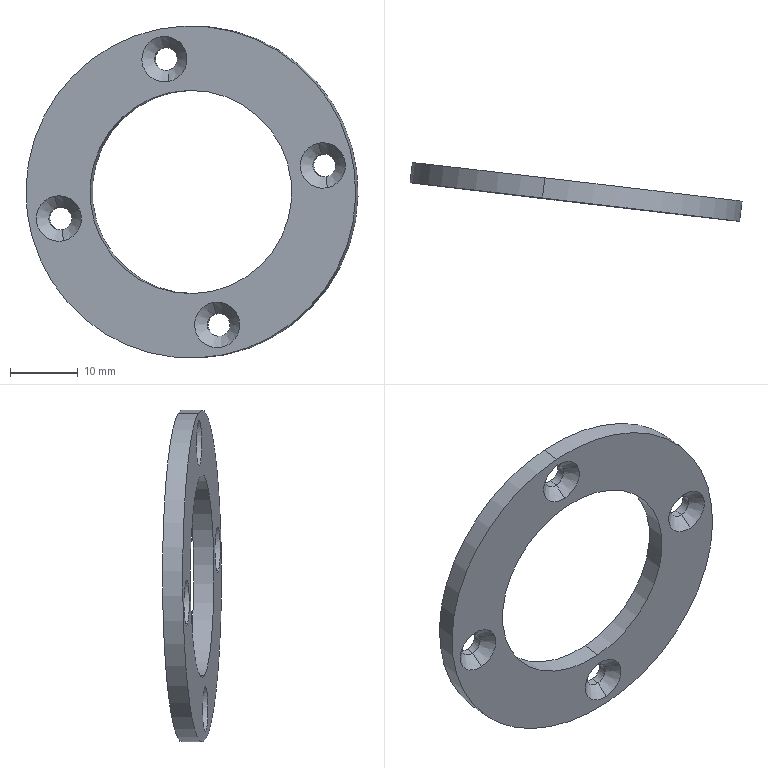Component | SolidWorks | 8TC-A17001-91-00UpperAndLowerPressAssembly-1_8TC-A17001-91-03Gland-1 | 1 solid | 22 faces | box 49.02 x 8.7 x 49 mm | volume 3350 mm3 | cylinder 12 | cone 8 | plane 2 | commonest cylinder face diameters 3.4 x8 30 x2 49 x2 | material A3
STEP:
#1=COLOUR_RGB('',0.7922,0.8196,0.9333);
#2=FILL_AREA_STYLE_COLOUR('',#1);
#3=FILL_AREA_STYLE('',(#2));
#4=SURFACE_STYLE_FILL_AREA(#3);
#5=SURFACE_SIDE_STYLE('',(#4));
#6=SURFACE_STYLE_USAGE(.BOTH.,#5);
#7=PRESENTATION_STYLE_ASSIGNMENT((#6));
#8=CARTESIAN_POINT('',(0.1834,-3.281,-2.754));
#9=VERTEX_POINT('',#8);
#10=CARTESIAN_POINT('',(0.2095,-3.284,-2.885));
#11=VERTEX_POINT('',#10);
#12=CARTESIAN_POINT('',(0.1964,-3.282,-2.819));
#13=DIRECTION('',(-0.1167,-0.9932,0.));
#14=DIRECTION('',(0.1946,-0.02286,-0.9806));
#15=AXIS2_PLACEMENT_3D('',#12,#13,#14);
#16=CIRCLE('',#15,0.06693);
#17=EDGE_CURVE('',#9,#11,#16,.T.);
#18=ORIENTED_EDGE('',*,*,#17,.F.);
#19=CARTESIAN_POINT('',(0.1631,-3.344,-2.69));
#20=VERTEX_POINT('',#19);
#21=CARTESIAN_POINT('',(0.1631,-3.344,-2.69));
#22=DIRECTION('',(-0.2201,-0.6861,0.6934));
#23=VECTOR('',#22,39.37);
#24=LINE('',#21,#23);
#25=EDGE_CURVE('',#9,#20,#24,.T.);
#26=ORIENTED_EDGE('',*,*,#25,.T.);
#27=CARTESIAN_POINT('',(0.2145,-3.35,-2.949));
#28=VERTEX_POINT('',#27);
#29=CARTESIAN_POINT('',(0.1888,-3.347,-2.819));
#30=DIRECTION('',(-0.1167,-0.9932,0.));
#31=DIRECTION('',(0.1946,-0.02286,-0.9806));
#32=AXIS2_PLACEMENT_3D('',#29,#30,#31);
#33=CIRCLE('',#32,0.1323);
#34=EDGE_CURVE('',#20,#28,#33,.T.);
#35=ORIENTED_EDGE('',*,*,#34,.T.);
#36=CARTESIAN_POINT('',(0.2145,-3.35,-2.949));
#37=DIRECTION('',(0.05511,-0.7184,-0.6934));
#38=VECTOR('',#37,39.37);
#39=LINE('',#36,#38);
#40=EDGE_CURVE('',#11,#28,#39,.T.);
#41=ORIENTED_EDGE('',*,*,#40,.F.);
#42=EDGE_LOOP('',(#18,#26,#35,#41));
#43=FACE_OUTER_BOUND('',#42,.T.);
#44=CARTESIAN_POINT('',(0.1888,-3.347,-2.819));
#45=DIRECTION('',(-0.1167,-0.9932,0.));
#46=DIRECTION('',(0.1946,-0.02286,-0.9806));
#47=AXIS2_PLACEMENT_3D('',#44,#45,#46);
#48=CONICAL_SURFACE('',#47,0.1323,0.7854);
#49=ADVANCED_FACE('',(#43),#48,.F.);
#50=CARTESIAN_POINT('',(0.1896,-3.228,-2.754));
#51=VERTEX_POINT('',#50);
#52=CARTESIAN_POINT('',(0.2156,-3.232,-2.885));
#53=VERTEX_POINT('',#52);
#54=CARTESIAN_POINT('',(0.2026,-3.23,-2.819));
#55=DIRECTION('',(-0.1167,-0.9932,0.));
#56=DIRECTION('',(0.1946,-0.02286,-0.9806));
#57=AXIS2_PLACEMENT_3D('',#54,#55,#56);
#58=CIRCLE('',#57,0.06693);
#59=EDGE_CURVE('',#51,#53,#58,.T.);
#60=ORIENTED_EDGE('',*,*,#59,.F.);
#61=CARTESIAN_POINT('',(0.1758,-3.346,-2.754));
#62=DIRECTION('',(-0.1167,-0.9932,0.));
#63=VECTOR('',#62,39.37);
#64=LINE('',#61,#63);
#65=EDGE_CURVE('',#51,#9,#64,.T.);
#66=ORIENTED_EDGE('',*,*,#65,.T.);
#67=ORIENTED_EDGE('',*,*,#17,.T.);
#68=CARTESIAN_POINT('',(0.2018,-3.349,-2.885));
#69=DIRECTION('',(-0.1167,-0.9932,0.));
#70=VECTOR('',#69,39.37);
#71=LINE('',#68,#70);
#72=EDGE_CURVE('',#53,#11,#71,.T.);
#73=ORIENTED_EDGE('',*,*,#72,.F.);
#74=EDGE_LOOP('',(#60,#66,#67,#73));
#75=FACE_OUTER_BOUND('',#74,.T.);
#76=CARTESIAN_POINT('',(0.1888,-3.347,-2.819));
#77=DIRECTION('',(-0.1167,-0.9932,0.));
#78=DIRECTION('',(0.1946,-0.02286,-0.9806));
#79=AXIS2_PLACEMENT_3D('',#76,#77,#78);
#80=CYLINDRICAL_SURFACE('',#79,0.06693);
#81=ADVANCED_FACE('',(#75),#80,.F.);
#82=CARTESIAN_POINT('',(0.797,-3.353,-1.827));
#83=VERTEX_POINT('',#82);
#84=CARTESIAN_POINT('',(0.8231,-3.356,-1.959));
#85=VERTEX_POINT('',#84);
#86=CARTESIAN_POINT('',(0.8101,-3.355,-1.893));
#87=DIRECTION('',(-0.1167,-0.9932,0.));
#88=DIRECTION('',(0.1946,-0.02286,-0.9806));
#89=AXIS2_PLACEMENT_3D('',#86,#87,#88);
#90=CIRCLE('',#89,0.06693);
#91=EDGE_CURVE('',#83,#85,#90,.T.);
#92=ORIENTED_EDGE('',*,*,#91,.F.);
#93=CARTESIAN_POINT('',(0.7767,-3.416,-1.763));
#94=VERTEX_POINT('',#93);
#95=CARTESIAN_POINT('',(0.7767,-3.416,-1.763));
#96=DIRECTION('',(-0.2201,-0.6861,0.6934));
#97=VECTOR('',#96,39.37);
#98=LINE('',#95,#97);
#99=EDGE_CURVE('',#83,#94,#98,.T.);
#100=ORIENTED_EDGE('',*,*,#99,.T.);
#101=CARTESIAN_POINT('',(0.8282,-3.422,-2.023));
#102=VERTEX_POINT('',#101);
#103=CARTESIAN_POINT('',(0.8024,-3.419,-1.893));
#104=DIRECTION('',(-0.1167,-0.9932,0.));
#105=DIRECTION('',(0.1946,-0.02286,-0.9806));
#106=AXIS2_PLACEMENT_3D('',#103,#104,#105);
#107=CIRCLE('',#106,0.1323);
#108=EDGE_CURVE('',#94,#102,#107,.T.);
#109=ORIENTED_EDGE('',*,*,#108,.T.);
#110=CARTESIAN_POINT('',(0.8282,-3.422,-2.023));
#111=DIRECTION('',(0.05511,-0.7184,-0.6934));
#112=VECTOR('',#111,39.37);
#113=LINE('',#110,#112);
#114=EDGE_CURVE('',#85,#102,#113,.T.);
#115=ORIENTED_EDGE('',*,*,#114,.F.);
#116=EDGE_LOOP('',(#92,#100,#109,#115));
#117=FACE_OUTER_BOUND('',#116,.T.);
#118=CARTESIAN_POINT('',(0.8024,-3.419,-1.893));
#119=DIRECTION('',(-0.1167,-0.9932,0.));
#120=DIRECTION('',(0.1946,-0.02286,-0.9806));
#121=AXIS2_PLACEMENT_3D('',#118,#119,#120);
#122=CONICAL_SURFACE('',#121,0.1323,0.7854);
#123=ADVANCED_FACE('',(#117),#122,.F.);
#124=CARTESIAN_POINT('',(0.8032,-3.301,-1.827));
#125=VERTEX_POINT('',#124);
#126=CARTESIAN_POINT('',(0.8292,-3.304,-1.959));
#127=VERTEX_POINT('',#126);
#128=CARTESIAN_POINT('',(0.8162,-3.302,-1.893));
#129=DIRECTION('',(-0.1167,-0.9932,0.));
#130=DIRECTION('',(0.1946,-0.02286,-0.9806));
#131=AXIS2_PLACEMENT_3D('',#128,#129,#130);
#132=CIRCLE('',#131,0.06693);
#133=EDGE_CURVE('',#125,#127,#132,.T.);
#134=ORIENTED_EDGE('',*,*,#133,.F.);
#135=CARTESIAN_POINT('',(0.7894,-3.418,-1.827));
#136=DIRECTION('',(-0.1167,-0.9932,0.));
#137=VECTOR('',#136,39.37);
#138=LINE('',#135,#137);
#139=EDGE_CURVE('',#125,#83,#138,.T.);
#140=ORIENTED_EDGE('',*,*,#139,.T.);
#141=ORIENTED_EDGE('',*,*,#91,.T.);
#142=CARTESIAN_POINT('',(0.8155,-3.421,-1.959));
#143=DIRECTION('',(-0.1167,-0.9932,0.));
#144=VECTOR('',#143,39.37);
#145=LINE('',#142,#144);
#146=EDGE_CURVE('',#127,#85,#145,.T.);
#147=ORIENTED_EDGE('',*,*,#146,.F.);
#148=EDGE_LOOP('',(#134,#140,#141,#147));
#149=FACE_OUTER_BOUND('',#148,.T.);
#150=CARTESIAN_POINT('',(0.8024,-3.419,-1.893));
#151=DIRECTION('',(-0.1167,-0.9932,0.));
#152=DIRECTION('',(0.1946,-0.02286,-0.9806));
#153=AXIS2_PLACEMENT_3D('',#150,#151,#152);
#154=CYLINDRICAL_SURFACE('',#153,0.06693);
#155=ADVANCED_FACE('',(#149),#154,.F.);
#156=CARTESIAN_POINT('',(-0.1231,-3.245,-1.209));
#157=VERTEX_POINT('',#156);
#158=CARTESIAN_POINT('',(-0.09702,-3.248,-1.341));
#159=VERTEX_POINT('',#158);
#160=CARTESIAN_POINT('',(-0.11,-3.246,-1.275));
#161=DIRECTION('',(-0.1167,-0.9932,0.));
#162=DIRECTION('',(0.1946,-0.02286,-0.9806));
#163=AXIS2_PLACEMENT_3D('',#160,#161,#162);
#164=CIRCLE('',#163,0.06693);
#165=EDGE_CURVE('',#157,#159,#164,.T.);
#166=ORIENTED_EDGE('',*,*,#165,.F.);
#167=CARTESIAN_POINT('',(-0.1434,-3.308,-1.145));
#168=VERTEX_POINT('',#167);
#169=CARTESIAN_POINT('',(-0.1434,-3.308,-1.145));
#170=DIRECTION('',(-0.2201,-0.6861,0.6934));
#171=VECTOR('',#170,39.37);
#172=LINE('',#169,#171);
#173=EDGE_CURVE('',#157,#168,#172,.T.);
#174=ORIENTED_EDGE('',*,*,#173,.T.);
#175=CARTESIAN_POINT('',(-0.09192,-3.314,-1.405));
#176=VERTEX_POINT('',#175);
#177=CARTESIAN_POINT('',(-0.1177,-3.311,-1.275));
#178=DIRECTION('',(-0.1167,-0.9932,0.));
#179=DIRECTION('',(0.1946,-0.02286,-0.9806));
#180=AXIS2_PLACEMENT_3D('',#177,#178,#179);
#181=CIRCLE('',#180,0.1323);
#182=EDGE_CURVE('',#168,#176,#181,.T.);
#183=ORIENTED_EDGE('',*,*,#182,.T.);
#184=CARTESIAN_POINT('',(-0.09192,-3.314,-1.405));
#185=DIRECTION('',(0.05511,-0.7184,-0.6934));
#186=VECTOR('',#185,39.37);
#187=LINE('',#184,#186);
#188=EDGE_CURVE('',#159,#176,#187,.T.);
#189=ORIENTED_EDGE('',*,*,#188,.F.);
#190=EDGE_LOOP('',(#166,#174,#183,#189));
#191=FACE_OUTER_BOUND('',#190,.T.);
#192=CARTESIAN_POINT('',(-0.1177,-3.311,-1.275));
#193=DIRECTION('',(-0.1167,-0.9932,0.));
#194=DIRECTION('',(0.1946,-0.02286,-0.9806));
#195=AXIS2_PLACEMENT_3D('',#192,#193,#194);
#196=CONICAL_SURFACE('',#195,0.1323,0.7854);
#197=ADVANCED_FACE('',(#191),#196,.F.);
#198=CARTESIAN_POINT('',(-0.1169,-3.192,-1.209));
#199=VERTEX_POINT('',#198);
#200=CARTESIAN_POINT('',(-0.09086,-3.196,-1.341));
#201=VERTEX_POINT('',#200);
#202=CARTESIAN_POINT('',(-0.1039,-3.194,-1.275));
#203=DIRECTION('',(-0.1167,-0.9932,0.));
#204=DIRECTION('',(0.1946,-0.02286,-0.9806));
#205=AXIS2_PLACEMENT_3D('',#202,#203,#204);
#206=CIRCLE('',#205,0.06693);
#207=EDGE_CURVE('',#199,#201,#206,.T.);
#208=ORIENTED_EDGE('',*,*,#207,.F.);
#209=CARTESIAN_POINT('',(-0.1307,-3.31,-1.209));
#210=DIRECTION('',(-0.1167,-0.9932,0.));
#211=VECTOR('',#210,39.37);
#212=LINE('',#209,#211);
#213=EDGE_CURVE('',#199,#157,#212,.T.);
#214=ORIENTED_EDGE('',*,*,#213,.T.);
#215=ORIENTED_EDGE('',*,*,#165,.T.);
#216=CARTESIAN_POINT('',(-0.1046,-3.313,-1.341));
#217=DIRECTION('',(-0.1167,-0.9932,0.));
#218=VECTOR('',#217,39.37);
#219=LINE('',#216,#218);
#220=EDGE_CURVE('',#201,#159,#219,.T.);
#221=ORIENTED_EDGE('',*,*,#220,.F.);
#222=EDGE_LOOP('',(#208,#214,#215,#221));
#223=FACE_OUTER_BOUND('',#222,.T.);
#224=CARTESIAN_POINT('',(-0.1177,-3.311,-1.275));
#225=DIRECTION('',(-0.1167,-0.9932,0.));
#226=DIRECTION('',(0.1946,-0.02286,-0.9806));
#227=AXIS2_PLACEMENT_3D('',#224,#225,#226);
#228=CYLINDRICAL_SURFACE('',#227,0.06693);
#229=ADVANCED_FACE('',(#223),#228,.F.);
#230=CARTESIAN_POINT('',(-0.7367,-3.173,-2.136));
#231=VERTEX_POINT('',#230);
#232=CARTESIAN_POINT('',(-0.7106,-3.176,-2.267));
#233=VERTEX_POINT('',#232);
#234=CARTESIAN_POINT('',(-0.7237,-3.174,-2.202));
#235=DIRECTION('',(-0.1167,-0.9932,0.));
#236=DIRECTION('',(0.1946,-0.02286,-0.9806));
#237=AXIS2_PLACEMENT_3D('',#234,#235,#236);
#238=CIRCLE('',#237,0.06693);
#239=EDGE_CURVE('',#231,#233,#238,.T.);
#240=ORIENTED_EDGE('',*,*,#239,.F.);
#241=CARTESIAN_POINT('',(-0.757,-3.236,-2.072));
#242=VERTEX_POINT('',#241);
#243=CARTESIAN_POINT('',(-0.757,-3.236,-2.072));
#244=DIRECTION('',(-0.2201,-0.6861,0.6934));
#245=VECTOR('',#244,39.37);
#246=LINE('',#243,#245);
#247=EDGE_CURVE('',#231,#242,#246,.T.);
#248=ORIENTED_EDGE('',*,*,#247,.T.);
#249=CARTESIAN_POINT('',(-0.7056,-3.242,-2.331));
#250=VERTEX_POINT('',#249);
#251=CARTESIAN_POINT('',(-0.7313,-3.239,-2.202));
#252=DIRECTION('',(-0.1167,-0.9932,0.));
#253=DIRECTION('',(0.1946,-0.02286,-0.9806));
#254=AXIS2_PLACEMENT_3D('',#251,#252,#253);
#255=CIRCLE('',#254,0.1323);
#256=EDGE_CURVE('',#242,#250,#255,.T.);
#257=ORIENTED_EDGE('',*,*,#256,.T.);
#258=CARTESIAN_POINT('',(-0.7056,-3.242,-2.331));
#259=DIRECTION('',(0.05511,-0.7184,-0.6934));
#260=VECTOR('',#259,39.37);
#261=LINE('',#258,#260);
#262=EDGE_CURVE('',#233,#250,#261,.T.);
#263=ORIENTED_EDGE('',*,*,#262,.F.);
#264=EDGE_LOOP('',(#240,#248,#257,#263));
#265=FACE_OUTER_BOUND('',#264,.T.);
#266=CARTESIAN_POINT('',(-0.7313,-3.239,-2.202));
#267=DIRECTION('',(-0.1167,-0.9932,0.));
#268=DIRECTION('',(0.1946,-0.02286,-0.9806));
#269=AXIS2_PLACEMENT_3D('',#266,#267,#268);
#270=CONICAL_SURFACE('',#269,0.1323,0.7854);
#271=ADVANCED_FACE('',(#265),#270,.F.);
#272=CARTESIAN_POINT('',(-0.7305,-3.12,-2.136));
#273=VERTEX_POINT('',#272);
#274=CARTESIAN_POINT('',(-0.7045,-3.123,-2.267));
#275=VERTEX_POINT('',#274);
#276=CARTESIAN_POINT('',(-0.7175,-3.122,-2.202));
#277=DIRECTION('',(-0.1167,-0.9932,0.));
#278=DIRECTION('',(0.1946,-0.02286,-0.9806));
#279=AXIS2_PLACEMENT_3D('',#276,#277,#278);
#280=CIRCLE('',#279,0.06693);
#281=EDGE_CURVE('',#273,#275,#280,.T.);
#282=ORIENTED_EDGE('',*,*,#281,.F.);
#283=CARTESIAN_POINT('',(-0.7443,-3.238,-2.136));
#284=DIRECTION('',(-0.1167,-0.9932,0.));
#285=VECTOR('',#284,39.37);
#286=LINE('',#283,#285);
#287=EDGE_CURVE('',#273,#231,#286,.T.);
#288=ORIENTED_EDGE('',*,*,#287,.T.);
#289=ORIENTED_EDGE('',*,*,#239,.T.);
#290=CARTESIAN_POINT('',(-0.7183,-3.241,-2.267));
#291=DIRECTION('',(-0.1167,-0.9932,0.));
#292=VECTOR('',#291,39.37);
#293=LINE('',#290,#292);
#294=EDGE_CURVE('',#275,#233,#293,.T.);
#295=ORIENTED_EDGE('',*,*,#294,.F.);
#296=EDGE_LOOP('',(#282,#288,#289,#295));
#297=FACE_OUTER_BOUND('',#296,.T.);
#298=CARTESIAN_POINT('',(-0.7313,-3.239,-2.202));
#299=DIRECTION('',(-0.1167,-0.9932,0.));
#300=DIRECTION('',(0.1946,-0.02286,-0.9806));
#301=AXIS2_PLACEMENT_3D('',#298,#299,#300);
#302=CYLINDRICAL_SURFACE('',#301,0.06693);
#303=ADVANCED_FACE('',(#297),#302,.F.);
#304=CARTESIAN_POINT('',(0.1643,-3.226,-2.626));
#305=VERTEX_POINT('',#304);
#306=CARTESIAN_POINT('',(-0.06558,-3.199,-1.468));
#307=VERTEX_POINT('',#306);
#308=CARTESIAN_POINT('',(0.04935,-3.212,-2.047));
#309=DIRECTION('',(0.1167,0.9932,-0.));
#310=DIRECTION('',(-0.1946,0.02286,0.9806));
#311=AXIS2_PLACEMENT_3D('',#308,#309,#310);
#312=CIRCLE('',#311,0.5906);
#313=EDGE_CURVE('',#305,#307,#312,.T.);
#314=ORIENTED_EDGE('',*,*,#313,.T.);
#315=CARTESIAN_POINT('',(-0.07936,-3.316,-1.468));
#316=VERTEX_POINT('',#315);
#317=CARTESIAN_POINT('',(-0.06558,-3.199,-1.468));
#318=DIRECTION('',(-0.1167,-0.9932,0.));
#319=VECTOR('',#318,39.37);
#320=LINE('',#317,#319);
#321=EDGE_CURVE('',#307,#316,#320,.T.);
#322=ORIENTED_EDGE('',*,*,#321,.T.);
#323=CARTESIAN_POINT('',(0.1505,-3.343,-2.626));
#324=VERTEX_POINT('',#323);
#325=CARTESIAN_POINT('',(0.03557,-3.329,-2.047));
#326=DIRECTION('',(0.1167,0.9932,-0.));
#327=DIRECTION('',(-0.1946,0.02286,0.9806));
#328=AXIS2_PLACEMENT_3D('',#325,#326,#327);
#329=CIRCLE('',#328,0.5906);
#330=EDGE_CURVE('',#324,#316,#329,.T.);
#331=ORIENTED_EDGE('',*,*,#330,.F.);
#332=CARTESIAN_POINT('',(0.1643,-3.226,-2.626));
#333=DIRECTION('',(-0.1167,-0.9932,0.));
#334=VECTOR('',#333,39.37);
#335=LINE('',#332,#334);
#336=EDGE_CURVE('',#305,#324,#335,.T.);
#337=ORIENTED_EDGE('',*,*,#336,.F.);
#338=EDGE_LOOP('',(#314,#322,#331,#337));
#339=FACE_OUTER_BOUND('',#338,.T.);
#340=CARTESIAN_POINT('',(0.04935,-3.212,-2.047));
#341=DIRECTION('',(-0.1167,-0.9932,0.));
#342=DIRECTION('',(0.1946,-0.02286,-0.9806));
#343=AXIS2_PLACEMENT_3D('',#340,#341,#342);
#344=CYLINDRICAL_SURFACE('',#343,0.5906);
#345=ADVANCED_FACE('',(#339),#344,.F.);
#346=CARTESIAN_POINT('',(-0.1384,-3.19,-1.101));
#347=VERTEX_POINT('',#346);
#348=CARTESIAN_POINT('',(0.2371,-3.234,-2.993));
#349=VERTEX_POINT('',#348);
#350=CARTESIAN_POINT('',(0.04935,-3.212,-2.047));
#351=DIRECTION('',(0.1167,0.9932,-0.));
#352=DIRECTION('',(-0.1946,0.02286,0.9806));
#353=AXIS2_PLACEMENT_3D('',#350,#351,#352);
#354=CIRCLE('',#353,0.9646);
#355=EDGE_CURVE('',#347,#349,#354,.T.);
#356=ORIENTED_EDGE('',*,*,#355,.F.);
#357=CARTESIAN_POINT('',(-0.1521,-3.307,-1.101));
#358=VERTEX_POINT('',#357);
#359=CARTESIAN_POINT('',(-0.1384,-3.19,-1.101));
#360=DIRECTION('',(-0.1167,-0.9932,0.));
#361=VECTOR('',#360,39.37);
#362=LINE('',#359,#361);
#363=EDGE_CURVE('',#347,#358,#362,.T.);
#364=ORIENTED_EDGE('',*,*,#363,.T.);
#365=CARTESIAN_POINT('',(0.2233,-3.351,-2.993));
#366=VERTEX_POINT('',#365);
#367=CARTESIAN_POINT('',(0.03557,-3.329,-2.047));
#368=DIRECTION('',(0.1167,0.9932,-0.));
#369=DIRECTION('',(-0.1946,0.02286,0.9806));
#370=AXIS2_PLACEMENT_3D('',#367,#368,#369);
#371=CIRCLE('',#370,0.9646);
#372=EDGE_CURVE('',#358,#366,#371,.T.);
#373=ORIENTED_EDGE('',*,*,#372,.T.);
#374=CARTESIAN_POINT('',(0.2371,-3.234,-2.993));
#375=DIRECTION('',(-0.1167,-0.9932,0.));
#376=VECTOR('',#375,39.37);
#377=LINE('',#374,#376);
#378=EDGE_CURVE('',#349,#366,#377,.T.);
#379=ORIENTED_EDGE('',*,*,#378,.F.);
#380=EDGE_LOOP('',(#356,#364,#373,#379));
#381=FACE_OUTER_BOUND('',#380,.T.);
#382=CARTESIAN_POINT('',(0.04935,-3.212,-2.047));
#383=DIRECTION('',(-0.1167,-0.9932,0.));
#384=DIRECTION('',(0.1946,-0.02286,-0.9806));
#385=AXIS2_PLACEMENT_3D('',#382,#383,#384);
#386=CYLINDRICAL_SURFACE('',#385,0.9646);
#387=ADVANCED_FACE('',(#381),#386,.T.);
#388=CARTESIAN_POINT('',(0.2026,-3.23,-2.819));
#389=DIRECTION('',(-0.1167,-0.9932,0.));
#390=DIRECTION('',(0.1946,-0.02286,-0.9806));
#391=AXIS2_PLACEMENT_3D('',#388,#389,#390);
#392=CIRCLE('',#391,0.06693);
#393=EDGE_CURVE('',#53,#51,#392,.T.);
#394=ORIENTED_EDGE('',*,*,#393,.T.);
#395=ORIENTED_EDGE('',*,*,#59,.T.);
#396=EDGE_LOOP('',(#394,#395));
#397=FACE_BOUND('',#396,.T.);
#398=CARTESIAN_POINT('',(0.8162,-3.302,-1.893));
#399=DIRECTION('',(-0.1167,-0.9932,0.));
#400=DIRECTION('',(0.1946,-0.02286,-0.9806));
#401=AXIS2_PLACEMENT_3D('',#398,#399,#400);
#402=CIRCLE('',#401,0.06693);
#403=EDGE_CURVE('',#127,#125,#402,.T.);
#404=ORIENTED_EDGE('',*,*,#403,.T.);
#405=ORIENTED_EDGE('',*,*,#133,.T.);
#406=EDGE_LOOP('',(#404,#405));
#407=FACE_BOUND('',#406,.T.);
#408=CARTESIAN_POINT('',(-0.1039,-3.194,-1.275));
#409=DIRECTION('',(-0.1167,-0.9932,0.));
#410=DIRECTION('',(0.1946,-0.02286,-0.9806));
#411=AXIS2_PLACEMENT_3D('',#408,#409,#410);
#412=CIRCLE('',#411,0.06693);
#413=EDGE_CURVE('',#201,#199,#412,.T.);
#414=ORIENTED_EDGE('',*,*,#413,.T.);
#415=ORIENTED_EDGE('',*,*,#207,.T.);
#416=EDGE_LOOP('',(#414,#415));
#417=FACE_BOUND('',#416,.T.);
#418=CARTESIAN_POINT('',(-0.7175,-3.122,-2.202));
#419=DIRECTION('',(-0.1167,-0.9932,0.));
#420=DIRECTION('',(0.1946,-0.02286,-0.9806));
#421=AXIS2_PLACEMENT_3D('',#418,#419,#420);
#422=CIRCLE('',#421,0.06693);
#423=EDGE_CURVE('',#275,#273,#422,.T.);
#424=ORIENTED_EDGE('',*,*,#423,.T.);
#425=ORIENTED_EDGE('',*,*,#281,.T.);
#426=EDGE_LOOP('',(#424,#425));
#427=FACE_BOUND('',#426,.T.);
#428=CARTESIAN_POINT('',(0.04935,-3.212,-2.047));
#429=DIRECTION('',(0.1167,0.9932,-0.));
#430=DIRECTION('',(-0.1946,0.02286,0.9806));
#431=AXIS2_PLACEMENT_3D('',#428,#429,#430);
#432=CIRCLE('',#431,0.9646);
#433=EDGE_CURVE('',#349,#347,#432,.T.);
#434=ORIENTED_EDGE('',*,*,#433,.T.);
#435=ORIENTED_EDGE('',*,*,#355,.T.);
#436=EDGE_LOOP('',(#434,#435));
#437=FACE_OUTER_BOUND('',#436,.T.);
#438=ORIENTED_EDGE('',*,*,#313,.F.);
#439=CARTESIAN_POINT('',(0.04935,-3.212,-2.047));
#440=DIRECTION('',(0.1167,0.9932,-0.));
#441=DIRECTION('',(-0.1946,0.02286,0.9806));
#442=AXIS2_PLACEMENT_3D('',#439,#440,#441);
#443=CIRCLE('',#442,0.5906);
#444=EDGE_CURVE('',#307,#305,#443,.T.);
#445=ORIENTED_EDGE('',*,*,#444,.F.);
#446=EDGE_LOOP('',(#438,#445));
#447=FACE_BOUND('',#446,.T.);
#448=CARTESIAN_POINT('',(0.04935,-3.212,-2.047));
#449=DIRECTION('',(0.1167,0.9932,-0.));
#450=DIRECTION('',(-0.1946,0.02286,0.9806));
#451=AXIS2_PLACEMENT_3D('',#448,#449,#450);
#452=PLANE('',#451);
#453=ADVANCED_FACE('',(#397,#407,#417,#427,#437,#447),#452,.T.);
#454=CARTESIAN_POINT('',(0.1888,-3.347,-2.819));
#455=DIRECTION('',(-0.1167,-0.9932,0.));
#456=DIRECTION('',(0.1946,-0.02286,-0.9806));
#457=AXIS2_PLACEMENT_3D('',#454,#455,#456);
#458=CIRCLE('',#457,0.1323);
#459=EDGE_CURVE('',#28,#20,#458,.T.);
#460=ORIENTED_EDGE('',*,*,#459,.F.);
#461=ORIENTED_EDGE('',*,*,#34,.F.);
#462=EDGE_LOOP('',(#460,#461));
#463=FACE_BOUND('',#462,.T.);
#464=CARTESIAN_POINT('',(0.8024,-3.419,-1.893));
#465=DIRECTION('',(-0.1167,-0.9932,0.));
#466=DIRECTION('',(0.1946,-0.02286,-0.9806));
#467=AXIS2_PLACEMENT_3D('',#464,#465,#466);
#468=CIRCLE('',#467,0.1323);
#469=EDGE_CURVE('',#102,#94,#468,.T.);
#470=ORIENTED_EDGE('',*,*,#469,.F.);
#471=ORIENTED_EDGE('',*,*,#108,.F.);
#472=EDGE_LOOP('',(#470,#471));
#473=FACE_BOUND('',#472,.T.);
#474=CARTESIAN_POINT('',(-0.1177,-3.311,-1.275));
#475=DIRECTION('',(-0.1167,-0.9932,0.));
#476=DIRECTION('',(0.1946,-0.02286,-0.9806));
#477=AXIS2_PLACEMENT_3D('',#474,#475,#476);
#478=CIRCLE('',#477,0.1323);
#479=EDGE_CURVE('',#176,#168,#478,.T.);
#480=ORIENTED_EDGE('',*,*,#479,.F.);
#481=ORIENTED_EDGE('',*,*,#182,.F.);
#482=EDGE_LOOP('',(#480,#481));
#483=FACE_BOUND('',#482,.T.);
#484=CARTESIAN_POINT('',(-0.7313,-3.239,-2.202));
#485=DIRECTION('',(-0.1167,-0.9932,0.));
#486=DIRECTION('',(0.1946,-0.02286,-0.9806));
#487=AXIS2_PLACEMENT_3D('',#484,#485,#486);
#488=CIRCLE('',#487,0.1323);
#489=EDGE_CURVE('',#250,#242,#488,.T.);
#490=ORIENTED_EDGE('',*,*,#489,.F.);
#491=ORIENTED_EDGE('',*,*,#256,.F.);
#492=EDGE_LOOP('',(#490,#491));
#493=FACE_BOUND('',#492,.T.);
#494=CARTESIAN_POINT('',(0.03557,-3.329,-2.047));
#495=DIRECTION('',(0.1167,0.9932,-0.));
#496=DIRECTION('',(-0.1946,0.02286,0.9806));
#497=AXIS2_PLACEMENT_3D('',#494,#495,#496);
#498=CIRCLE('',#497,0.9646);
#499=EDGE_CURVE('',#366,#358,#498,.T.);
#500=ORIENTED_EDGE('',*,*,#499,.F.);
#501=ORIENTED_EDGE('',*,*,#372,.F.);
#502=EDGE_LOOP('',(#500,#501));
#503=FACE_OUTER_BOUND('',#502,.T.);
#504=ORIENTED_EDGE('',*,*,#330,.T.);
#505=CARTESIAN_POINT('',(0.03557,-3.329,-2.047));
#506=DIRECTION('',(0.1167,0.9932,-0.));
#507=DIRECTION('',(-0.1946,0.02286,0.9806));
#508=AXIS2_PLACEMENT_3D('',#505,#506,#507);
#509=CIRCLE('',#508,0.5906);
#510=EDGE_CURVE('',#316,#324,#509,.T.);
#511=ORIENTED_EDGE('',*,*,#510,.T.);
#512=EDGE_LOOP('',(#504,#511));
#513=FACE_BOUND('',#512,.T.);
#514=CARTESIAN_POINT('',(0.03557,-3.329,-2.047));
#515=DIRECTION('',(0.1167,0.9932,-0.));
#516=DIRECTION('',(-0.1946,0.02286,0.9806));
#517=AXIS2_PLACEMENT_3D('',#514,#515,#516);
#518=PLANE('',#517);
#519=ADVANCED_FACE('',(#463,#473,#483,#493,#503,#513),#518,.F.);
#520=ORIENTED_EDGE('',*,*,#363,.F.);
#521=ORIENTED_EDGE('',*,*,#433,.F.);
#522=ORIENTED_EDGE('',*,*,#378,.T.);
#523=ORIENTED_EDGE('',*,*,#499,.T.);
#524=EDGE_LOOP('',(#520,#521,#522,#523));
#525=FACE_OUTER_BOUND('',#524,.T.);
#526=CARTESIAN_POINT('',(0.04935,-3.212,-2.047));
#527=DIRECTION('',(-0.1167,-0.9932,0.));
#528=DIRECTION('',(0.1946,-0.02286,-0.9806));
#529=AXIS2_PLACEMENT_3D('',#526,#527,#528);
#530=CYLINDRICAL_SURFACE('',#529,0.9646);
#531=ADVANCED_FACE('',(#525),#530,.T.);
#532=ORIENTED_EDGE('',*,*,#321,.F.);
#533=ORIENTED_EDGE('',*,*,#444,.T.);
#534=ORIENTED_EDGE('',*,*,#336,.T.);
#535=ORIENTED_EDGE('',*,*,#510,.F.);
#536=EDGE_LOOP('',(#532,#533,#534,#535));
#537=FACE_OUTER_BOUND('',#536,.T.);
#538=CARTESIAN_POINT('',(0.04935,-3.212,-2.047));
#539=DIRECTION('',(-0.1167,-0.9932,0.));
#540=DIRECTION('',(0.1946,-0.02286,-0.9806));
#541=AXIS2_PLACEMENT_3D('',#538,#539,#540);
#542=CYLINDRICAL_SURFACE('',#541,0.5906);
#543=ADVANCED_FACE('',(#537),#542,.F.);
#544=ORIENTED_EDGE('',*,*,#287,.F.);
#545=ORIENTED_EDGE('',*,*,#423,.F.);
#546=ORIENTED_EDGE('',*,*,#294,.T.);
#547=CARTESIAN_POINT('',(-0.7237,-3.174,-2.202));
#548=DIRECTION('',(-0.1167,-0.9932,0.));
#549=DIRECTION('',(0.1946,-0.02286,-0.9806));
#550=AXIS2_PLACEMENT_3D('',#547,#548,#549);
#551=CIRCLE('',#550,0.06693);
#552=EDGE_CURVE('',#233,#231,#551,.T.);
#553=ORIENTED_EDGE('',*,*,#552,.T.);
#554=EDGE_LOOP('',(#544,#545,#546,#553));
#555=FACE_OUTER_BOUND('',#554,.T.);
#556=CARTESIAN_POINT('',(-0.7313,-3.239,-2.202));
#557=DIRECTION('',(-0.1167,-0.9932,0.));
#558=DIRECTION('',(0.1946,-0.02286,-0.9806));
#559=AXIS2_PLACEMENT_3D('',#556,#557,#558);
#560=CYLINDRICAL_SURFACE('',#559,0.06693);
#561=ADVANCED_FACE('',(#555),#560,.F.);
#562=ORIENTED_EDGE('',*,*,#247,.F.);
#563=ORIENTED_EDGE('',*,*,#552,.F.);
#564=ORIENTED_EDGE('',*,*,#262,.T.);
#565=ORIENTED_EDGE('',*,*,#489,.T.);
#566=EDGE_LOOP('',(#562,#563,#564,#565));
#567=FACE_OUTER_BOUND('',#566,.T.);
#568=CARTESIAN_POINT('',(-0.7313,-3.239,-2.202));
#569=DIRECTION('',(-0.1167,-0.9932,0.));
#570=DIRECTION('',(0.1946,-0.02286,-0.9806));
#571=AXIS2_PLACEMENT_3D('',#568,#569,#570);
#572=CONICAL_SURFACE('',#571,0.1323,0.7854);
#573=ADVANCED_FACE('',(#567),#572,.F.);
#574=ORIENTED_EDGE('',*,*,#213,.F.);
#575=ORIENTED_EDGE('',*,*,#413,.F.);
#576=ORIENTED_EDGE('',*,*,#220,.T.);
#577=CARTESIAN_POINT('',(-0.11,-3.246,-1.275));
#578=DIRECTION('',(-0.1167,-0.9932,0.));
#579=DIRECTION('',(0.1946,-0.02286,-0.9806));
#580=AXIS2_PLACEMENT_3D('',#577,#578,#579);
#581=CIRCLE('',#580,0.06693);
#582=EDGE_CURVE('',#159,#157,#581,.T.);
#583=ORIENTED_EDGE('',*,*,#582,.T.);
#584=EDGE_LOOP('',(#574,#575,#576,#583));
#585=FACE_OUTER_BOUND('',#584,.T.);
#586=CARTESIAN_POINT('',(-0.1177,-3.311,-1.275));
#587=DIRECTION('',(-0.1167,-0.9932,0.));
#588=DIRECTION('',(0.1946,-0.02286,-0.9806));
#589=AXIS2_PLACEMENT_3D('',#586,#587,#588);
#590=CYLINDRICAL_SURFACE('',#589,0.06693);
#591=ADVANCED_FACE('',(#585),#590,.F.);
#592=ORIENTED_EDGE('',*,*,#173,.F.);
#593=ORIENTED_EDGE('',*,*,#582,.F.);
#594=ORIENTED_EDGE('',*,*,#188,.T.);
#595=ORIENTED_EDGE('',*,*,#479,.T.);
#596=EDGE_LOOP('',(#592,#593,#594,#595));
#597=FACE_OUTER_BOUND('',#596,.T.);
#598=CARTESIAN_POINT('',(-0.1177,-3.311,-1.275));
#599=DIRECTION('',(-0.1167,-0.9932,0.));
#600=DIRECTION('',(0.1946,-0.02286,-0.9806));
#601=AXIS2_PLACEMENT_3D('',#598,#599,#600);
#602=CONICAL_SURFACE('',#601,0.1323,0.7854);
#603=ADVANCED_FACE('',(#597),#602,.F.);
#604=ORIENTED_EDGE('',*,*,#139,.F.);
#605=ORIENTED_EDGE('',*,*,#403,.F.);
#606=ORIENTED_EDGE('',*,*,#146,.T.);
#607=CARTESIAN_POINT('',(0.8101,-3.355,-1.893));
#608=DIRECTION('',(-0.1167,-0.9932,0.));
#609=DIRECTION('',(0.1946,-0.02286,-0.9806));
#610=AXIS2_PLACEMENT_3D('',#607,#608,#609);
#611=CIRCLE('',#610,0.06693);
#612=EDGE_CURVE('',#85,#83,#611,.T.);
#613=ORIENTED_EDGE('',*,*,#612,.T.);
#614=EDGE_LOOP('',(#604,#605,#606,#613));
#615=FACE_OUTER_BOUND('',#614,.T.);
#616=CARTESIAN_POINT('',(0.8024,-3.419,-1.893));
#617=DIRECTION('',(-0.1167,-0.9932,0.));
#618=DIRECTION('',(0.1946,-0.02286,-0.9806));
#619=AXIS2_PLACEMENT_3D('',#616,#617,#618);
#620=CYLINDRICAL_SURFACE('',#619,0.06693);
#621=ADVANCED_FACE('',(#615),#620,.F.);
#622=ORIENTED_EDGE('',*,*,#99,.F.);
#623=ORIENTED_EDGE('',*,*,#612,.F.);
#624=ORIENTED_EDGE('',*,*,#114,.T.);
#625=ORIENTED_EDGE('',*,*,#469,.T.);
#626=EDGE_LOOP('',(#622,#623,#624,#625));
#627=FACE_OUTER_BOUND('',#626,.T.);
#628=CARTESIAN_POINT('',(0.8024,-3.419,-1.893));
#629=DIRECTION('',(-0.1167,-0.9932,0.));
#630=DIRECTION('',(0.1946,-0.02286,-0.9806));
#631=AXIS2_PLACEMENT_3D('',#628,#629,#630);
#632=CONICAL_SURFACE('',#631,0.1323,0.7854);
#633=ADVANCED_FACE('',(#627),#632,.F.);
#634=ORIENTED_EDGE('',*,*,#65,.F.);
#635=ORIENTED_EDGE('',*,*,#393,.F.);
#636=ORIENTED_EDGE('',*,*,#72,.T.);
#637=CARTESIAN_POINT('',(0.1964,-3.282,-2.819));
#638=DIRECTION('',(-0.1167,-0.9932,0.));
#639=DIRECTION('',(0.1946,-0.02286,-0.9806));
#640=AXIS2_PLACEMENT_3D('',#637,#638,#639);
#641=CIRCLE('',#640,0.06693);
#642=EDGE_CURVE('',#11,#9,#641,.T.);
#643=ORIENTED_EDGE('',*,*,#642,.T.);
#644=EDGE_LOOP('',(#634,#635,#636,#643));
#645=FACE_OUTER_BOUND('',#644,.T.);
#646=CARTESIAN_POINT('',(0.1888,-3.347,-2.819));
#647=DIRECTION('',(-0.1167,-0.9932,0.));
#648=DIRECTION('',(0.1946,-0.02286,-0.9806));
#649=AXIS2_PLACEMENT_3D('',#646,#647,#648);
#650=CYLINDRICAL_SURFACE('',#649,0.06693);
#651=ADVANCED_FACE('',(#645),#650,.F.);
#652=ORIENTED_EDGE('',*,*,#25,.F.);
#653=ORIENTED_EDGE('',*,*,#642,.F.);
#654=ORIENTED_EDGE('',*,*,#40,.T.);
#655=ORIENTED_EDGE('',*,*,#459,.T.);
#656=EDGE_LOOP('',(#652,#653,#654,#655));
#657=FACE_OUTER_BOUND('',#656,.T.);
#658=CARTESIAN_POINT('',(0.1888,-3.347,-2.819));
#659=DIRECTION('',(-0.1167,-0.9932,0.));
#660=DIRECTION('',(0.1946,-0.02286,-0.9806));
#661=AXIS2_PLACEMENT_3D('',#658,#659,#660);
#662=CONICAL_SURFACE('',#661,0.1323,0.7854);
#663=ADVANCED_FACE('',(#657),#662,.F.);
#664=CLOSED_SHELL('',(#49,#81,#123,#155,#197,#229,#271,#303,#345,#387,#453,#519,#531,#543,#561,#573,#591,#603,#621,#633,#651,#663));
#665=MANIFOLD_SOLID_BREP('',#664);
#666=STYLED_ITEM('',(#7),#665);
#667=PRESENTATION_LAYER_ASSIGNMENT('','',(#666));
#668=CARTESIAN_POINT('',(0.,0.,0.));
#669=DIRECTION('',(0.,0.,1.));
#670=DIRECTION('',(1.,0.,0.));
#671=AXIS2_PLACEMENT_3D('',#668,#669,#670);
#672=(LENGTH_UNIT()NAMED_UNIT(*)SI_UNIT($,.METRE.));
#673=LENGTH_MEASURE_WITH_UNIT(LENGTH_MEASURE(0.0254),#672);
#674=DIMENSIONAL_EXPONENTS(1.,0.,0.,0.,0.,0.,0.);
#675=(CONVERSION_BASED_UNIT('',#673)LENGTH_UNIT()NAMED_UNIT(#674));
#676=UNCERTAINTY_MEASURE_WITH_UNIT(LENGTH_MEASURE(0.00001),#675,'','');
#677=(NAMED_UNIT(*)PLANE_ANGLE_UNIT()SI_UNIT($,.RADIAN.));
#678=(NAMED_UNIT(*)SI_UNIT($,.STERADIAN.)SOLID_ANGLE_UNIT());
#679=(GEOMETRIC_REPRESENTATION_CONTEXT(3)GLOBAL_UNCERTAINTY_ASSIGNED_CONTEXT((#676))GLOBAL_UNIT_ASSIGNED_CONTEXT((#675,#677,#678))REPRESENTATION_CONTEXT('',''));
#680=ADVANCED_BREP_SHAPE_REPRESENTATION('',(#665,#671),#679);
#681=(LENGTH_UNIT()NAMED_UNIT(*)SI_UNIT($,.METRE.));
#682=LENGTH_MEASURE_WITH_UNIT(LENGTH_MEASURE(0.0254),#681);
#683=DIMENSIONAL_EXPONENTS(1.,0.,0.,0.,0.,0.,0.);
#684=(CONVERSION_BASED_UNIT('',#682)LENGTH_UNIT()NAMED_UNIT(#683));
#685=UNCERTAINTY_MEASURE_WITH_UNIT(LENGTH_MEASURE(0.00001),#684,'','');
#686=(NAMED_UNIT(*)PLANE_ANGLE_UNIT()SI_UNIT($,.RADIAN.));
#687=(NAMED_UNIT(*)SI_UNIT($,.STERADIAN.)SOLID_ANGLE_UNIT());
#688=(GEOMETRIC_REPRESENTATION_CONTEXT(3)GLOBAL_UNCERTAINTY_ASSIGNED_CONTEXT((#685))GLOBAL_UNIT_ASSIGNED_CONTEXT((#684,#686,#687))REPRESENTATION_CONTEXT('',''));
#689=MECHANICAL_DESIGN_GEOMETRIC_PRESENTATION_REPRESENTATION('',(#666),#688);